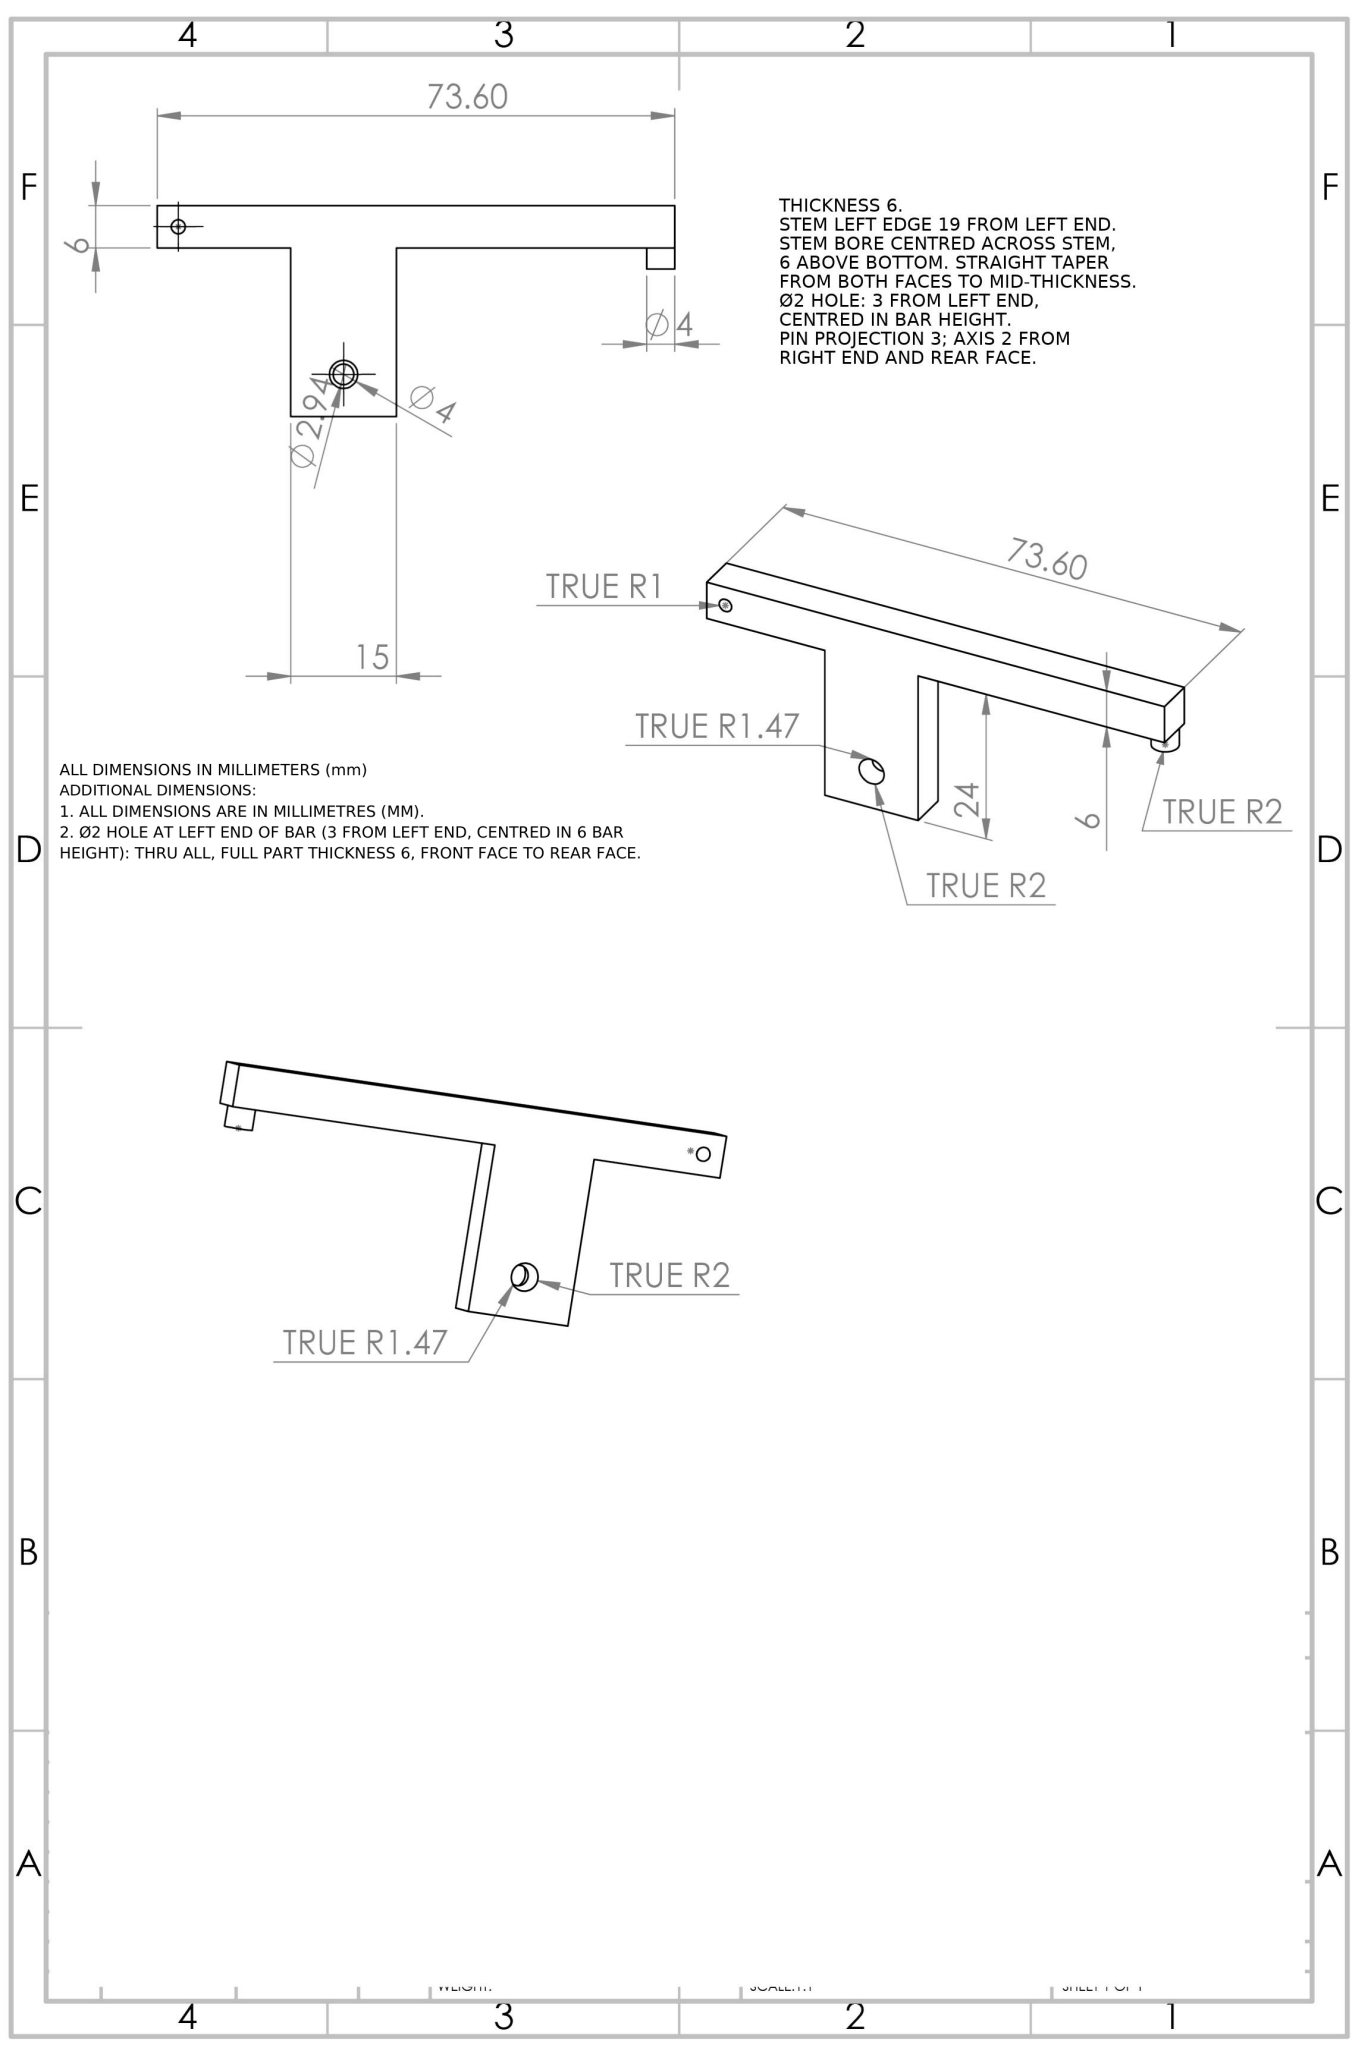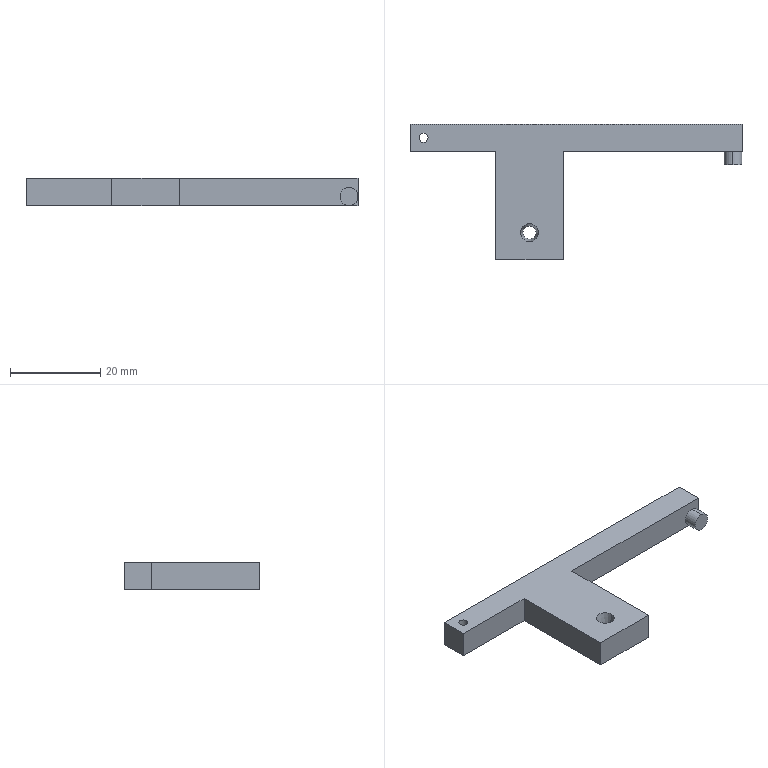Part | NX | mm | Z-Shaped Boss Link Bracket | 1 solid | 20 faces | box 73.6 x 30 x 6 mm | volume 4771 mm3 | plane 12 | cylinder 4 | cone 4 | commonest cylinder face diameters 4 x2 2 x2
STEP:
#1=COLOUR_RGB('',0.6706,0.8667,1.);
#2=FILL_AREA_STYLE_COLOUR('',#1);
#3=FILL_AREA_STYLE('',(#2));
#4=SURFACE_STYLE_FILL_AREA(#3);
#5=SURFACE_SIDE_STYLE('',(#4));
#6=SURFACE_STYLE_USAGE(.BOTH.,#5);
#7=PRESENTATION_STYLE_ASSIGNMENT((#6));
#8=CARTESIAN_POINT('',(2.,-9.,-0.));
#9=VERTEX_POINT('',#8);
#10=CARTESIAN_POINT('',(2.,-9.,4.));
#11=VERTEX_POINT('',#10);
#12=CARTESIAN_POINT('',(2.,-9.,2.));
#13=DIRECTION('',(0.,-1.,0.));
#14=DIRECTION('',(0.,0.,-1.));
#15=AXIS2_PLACEMENT_3D('',#12,#13,#14);
#16=CIRCLE('',#15,2.);
#17=EDGE_CURVE('',#9,#11,#16,.T.);
#18=ORIENTED_EDGE('',*,*,#17,.F.);
#19=CARTESIAN_POINT('',(2.,-6.,0.));
#20=VERTEX_POINT('',#19);
#21=CARTESIAN_POINT('',(2.,-9.,-0.));
#22=DIRECTION('',(0.,1.,0.));
#23=VECTOR('',#22,1000.);
#24=LINE('',#21,#23);
#25=EDGE_CURVE('',#9,#20,#24,.T.);
#26=ORIENTED_EDGE('',*,*,#25,.T.);
#27=CARTESIAN_POINT('',(4.,-6.,2.));
#28=VERTEX_POINT('',#27);
#29=CARTESIAN_POINT('',(2.,-6.,2.));
#30=DIRECTION('',(0.,-1.,0.));
#31=DIRECTION('',(0.,0.,-1.));
#32=AXIS2_PLACEMENT_3D('',#29,#30,#31);
#33=CIRCLE('',#32,2.);
#34=EDGE_CURVE('',#20,#28,#33,.T.);
#35=ORIENTED_EDGE('',*,*,#34,.T.);
#36=CARTESIAN_POINT('',(2.,-6.,4.));
#37=VERTEX_POINT('',#36);
#38=CARTESIAN_POINT('',(2.,-6.,2.));
#39=DIRECTION('',(0.,-1.,0.));
#40=DIRECTION('',(0.,0.,-1.));
#41=AXIS2_PLACEMENT_3D('',#38,#39,#40);
#42=CIRCLE('',#41,2.);
#43=EDGE_CURVE('',#28,#37,#42,.T.);
#44=ORIENTED_EDGE('',*,*,#43,.T.);
#45=CARTESIAN_POINT('',(2.,-9.,4.));
#46=DIRECTION('',(0.,1.,0.));
#47=VECTOR('',#46,1000.);
#48=LINE('',#45,#47);
#49=EDGE_CURVE('',#11,#37,#48,.T.);
#50=ORIENTED_EDGE('',*,*,#49,.F.);
#51=EDGE_LOOP('',(#18,#26,#35,#44,#50));
#52=FACE_OUTER_BOUND('',#51,.T.);
#53=CARTESIAN_POINT('',(2.,-9.,2.));
#54=DIRECTION('',(0.,1.,0.));
#55=DIRECTION('',(0.,0.,1.));
#56=AXIS2_PLACEMENT_3D('',#53,#54,#55);
#57=CYLINDRICAL_SURFACE('',#56,2.);
#58=ADVANCED_FACE('',(#52),#57,.T.);
#59=CARTESIAN_POINT('',(-67.6,-3.,0.));
#60=VERTEX_POINT('',#59);
#61=CARTESIAN_POINT('',(-65.6,-3.,0.));
#62=VERTEX_POINT('',#61);
#63=CARTESIAN_POINT('',(-66.6,-3.,0.));
#64=DIRECTION('',(0.,0.,1.));
#65=DIRECTION('',(1.,0.,0.));
#66=AXIS2_PLACEMENT_3D('',#63,#64,#65);
#67=CIRCLE('',#66,1.);
#68=EDGE_CURVE('',#60,#62,#67,.T.);
#69=ORIENTED_EDGE('',*,*,#68,.F.);
#70=CARTESIAN_POINT('',(-67.6,-3.,6.));
#71=VERTEX_POINT('',#70);
#72=CARTESIAN_POINT('',(-67.6,-3.,0.));
#73=DIRECTION('',(0.,0.,1.));
#74=VECTOR('',#73,1000.);
#75=LINE('',#72,#74);
#76=EDGE_CURVE('',#60,#71,#75,.T.);
#77=ORIENTED_EDGE('',*,*,#76,.T.);
#78=CARTESIAN_POINT('',(-65.6,-3.,6.));
#79=VERTEX_POINT('',#78);
#80=CARTESIAN_POINT('',(-66.6,-3.,6.));
#81=DIRECTION('',(0.,0.,1.));
#82=DIRECTION('',(1.,0.,0.));
#83=AXIS2_PLACEMENT_3D('',#80,#81,#82);
#84=CIRCLE('',#83,1.);
#85=EDGE_CURVE('',#71,#79,#84,.T.);
#86=ORIENTED_EDGE('',*,*,#85,.T.);
#87=CARTESIAN_POINT('',(-65.6,-3.,0.));
#88=DIRECTION('',(0.,0.,1.));
#89=VECTOR('',#88,1000.);
#90=LINE('',#87,#89);
#91=EDGE_CURVE('',#62,#79,#90,.T.);
#92=ORIENTED_EDGE('',*,*,#91,.F.);
#93=EDGE_LOOP('',(#69,#77,#86,#92));
#94=FACE_OUTER_BOUND('',#93,.T.);
#95=CARTESIAN_POINT('',(-66.6,-3.,0.));
#96=DIRECTION('',(0.,0.,1.));
#97=DIRECTION('',(1.,0.,0.));
#98=AXIS2_PLACEMENT_3D('',#95,#96,#97);
#99=CYLINDRICAL_SURFACE('',#98,1.);
#100=ADVANCED_FACE('',(#94),#99,.F.);
#101=CARTESIAN_POINT('',(-41.629,-24.,3.));
#102=VERTEX_POINT('',#101);
#103=CARTESIAN_POINT('',(-44.571,-24.,3.));
#104=VERTEX_POINT('',#103);
#105=CARTESIAN_POINT('',(-43.1,-24.,3.));
#106=DIRECTION('',(0.,0.,-1.));
#107=DIRECTION('',(-1.,0.,0.));
#108=AXIS2_PLACEMENT_3D('',#105,#106,#107);
#109=CIRCLE('',#108,1.471);
#110=EDGE_CURVE('',#102,#104,#109,.T.);
#111=ORIENTED_EDGE('',*,*,#110,.F.);
#112=CARTESIAN_POINT('',(-41.1,-24.,0.));
#113=VERTEX_POINT('',#112);
#114=CARTESIAN_POINT('',(-41.1,-24.,0.));
#115=DIRECTION('',(0.1736,0.,-0.9848));
#116=VECTOR('',#115,1000.);
#117=LINE('',#114,#116);
#118=EDGE_CURVE('',#102,#113,#117,.T.);
#119=ORIENTED_EDGE('',*,*,#118,.T.);
#120=CARTESIAN_POINT('',(-45.1,-24.,0.));
#121=VERTEX_POINT('',#120);
#122=CARTESIAN_POINT('',(-43.1,-24.,0.));
#123=DIRECTION('',(0.,0.,-1.));
#124=DIRECTION('',(-1.,0.,0.));
#125=AXIS2_PLACEMENT_3D('',#122,#123,#124);
#126=CIRCLE('',#125,2.);
#127=EDGE_CURVE('',#113,#121,#126,.T.);
#128=ORIENTED_EDGE('',*,*,#127,.T.);
#129=CARTESIAN_POINT('',(-45.1,-24.,0.));
#130=DIRECTION('',(-0.1736,0.,-0.9848));
#131=VECTOR('',#130,1000.);
#132=LINE('',#129,#131);
#133=EDGE_CURVE('',#104,#121,#132,.T.);
#134=ORIENTED_EDGE('',*,*,#133,.F.);
#135=EDGE_LOOP('',(#111,#119,#128,#134));
#136=FACE_OUTER_BOUND('',#135,.T.);
#137=CARTESIAN_POINT('',(-43.1,-24.,0.));
#138=DIRECTION('',(0.,0.,-1.));
#139=DIRECTION('',(-1.,0.,0.));
#140=AXIS2_PLACEMENT_3D('',#137,#138,#139);
#141=CONICAL_SURFACE('',#140,2.,0.1745);
#142=ADVANCED_FACE('',(#136),#141,.F.);
#143=ORIENTED_EDGE('',*,*,#110,.T.);
#144=CARTESIAN_POINT('',(-45.1,-24.,6.));
#145=VERTEX_POINT('',#144);
#146=CARTESIAN_POINT('',(-45.1,-24.,6.));
#147=DIRECTION('',(-0.1736,0.,0.9848));
#148=VECTOR('',#147,1000.);
#149=LINE('',#146,#148);
#150=EDGE_CURVE('',#104,#145,#149,.T.);
#151=ORIENTED_EDGE('',*,*,#150,.T.);
#152=CARTESIAN_POINT('',(-41.1,-24.,6.));
#153=VERTEX_POINT('',#152);
#154=CARTESIAN_POINT('',(-43.1,-24.,6.));
#155=DIRECTION('',(0.,0.,1.));
#156=DIRECTION('',(1.,0.,0.));
#157=AXIS2_PLACEMENT_3D('',#154,#155,#156);
#158=CIRCLE('',#157,2.);
#159=EDGE_CURVE('',#145,#153,#158,.T.);
#160=ORIENTED_EDGE('',*,*,#159,.T.);
#161=CARTESIAN_POINT('',(-41.1,-24.,6.));
#162=DIRECTION('',(0.1736,0.,0.9848));
#163=VECTOR('',#162,1000.);
#164=LINE('',#161,#163);
#165=EDGE_CURVE('',#102,#153,#164,.T.);
#166=ORIENTED_EDGE('',*,*,#165,.F.);
#167=EDGE_LOOP('',(#143,#151,#160,#166));
#168=FACE_OUTER_BOUND('',#167,.T.);
#169=CARTESIAN_POINT('',(-43.1,-24.,6.));
#170=DIRECTION('',(0.,0.,1.));
#171=DIRECTION('',(1.,0.,0.));
#172=AXIS2_PLACEMENT_3D('',#169,#170,#171);
#173=CONICAL_SURFACE('',#172,2.,0.1745);
#174=ADVANCED_FACE('',(#168),#173,.F.);
#175=ORIENTED_EDGE('',*,*,#34,.F.);
#176=CARTESIAN_POINT('',(4.,-6.,0.));
#177=VERTEX_POINT('',#176);
#178=CARTESIAN_POINT('',(0.,-6.,0.));
#179=DIRECTION('',(1.,0.,0.));
#180=VECTOR('',#179,1000.);
#181=LINE('',#178,#180);
#182=EDGE_CURVE('',#20,#177,#181,.T.);
#183=ORIENTED_EDGE('',*,*,#182,.T.);
#184=CARTESIAN_POINT('',(4.,-6.,6.));
#185=DIRECTION('',(0.,0.,-1.));
#186=VECTOR('',#185,1000.);
#187=LINE('',#184,#186);
#188=EDGE_CURVE('',#28,#177,#187,.T.);
#189=ORIENTED_EDGE('',*,*,#188,.F.);
#190=EDGE_LOOP('',(#175,#183,#189));
#191=FACE_OUTER_BOUND('',#190,.T.);
#192=CARTESIAN_POINT('',(0.,-6.,6.));
#193=DIRECTION('',(0.,1.,0.));
#194=DIRECTION('',(0.,0.,1.));
#195=AXIS2_PLACEMENT_3D('',#192,#193,#194);
#196=PLANE('',#195);
#197=ADVANCED_FACE('',(#191),#196,.F.);
#198=CARTESIAN_POINT('',(4.,-0.,0.));
#199=VERTEX_POINT('',#198);
#200=CARTESIAN_POINT('',(-69.6,-0.,0.));
#201=VERTEX_POINT('',#200);
#202=CARTESIAN_POINT('',(-69.6,-0.,0.));
#203=DIRECTION('',(-1.,-0.,0.));
#204=VECTOR('',#203,1000.);
#205=LINE('',#202,#204);
#206=EDGE_CURVE('',#199,#201,#205,.T.);
#207=ORIENTED_EDGE('',*,*,#206,.T.);
#208=CARTESIAN_POINT('',(-69.6,-0.,6.));
#209=VERTEX_POINT('',#208);
#210=CARTESIAN_POINT('',(-69.6,-0.,6.));
#211=DIRECTION('',(0.,0.,-1.));
#212=VECTOR('',#211,1000.);
#213=LINE('',#210,#212);
#214=EDGE_CURVE('',#209,#201,#213,.T.);
#215=ORIENTED_EDGE('',*,*,#214,.F.);
#216=CARTESIAN_POINT('',(4.,-0.,6.));
#217=VERTEX_POINT('',#216);
#218=CARTESIAN_POINT('',(-69.6,-0.,6.));
#219=DIRECTION('',(-1.,-0.,0.));
#220=VECTOR('',#219,1000.);
#221=LINE('',#218,#220);
#222=EDGE_CURVE('',#217,#209,#221,.T.);
#223=ORIENTED_EDGE('',*,*,#222,.F.);
#224=CARTESIAN_POINT('',(4.,-0.,6.));
#225=DIRECTION('',(0.,0.,-1.));
#226=VECTOR('',#225,1000.);
#227=LINE('',#224,#226);
#228=EDGE_CURVE('',#217,#199,#227,.T.);
#229=ORIENTED_EDGE('',*,*,#228,.T.);
#230=EDGE_LOOP('',(#207,#215,#223,#229));
#231=FACE_OUTER_BOUND('',#230,.T.);
#232=CARTESIAN_POINT('',(-69.6,-0.,6.));
#233=DIRECTION('',(0.,-1.,0.));
#234=DIRECTION('',(1.,0.,0.));
#235=AXIS2_PLACEMENT_3D('',#232,#233,#234);
#236=PLANE('',#235);
#237=ADVANCED_FACE('',(#231),#236,.F.);
#238=CARTESIAN_POINT('',(-69.6,-6.,0.));
#239=VERTEX_POINT('',#238);
#240=CARTESIAN_POINT('',(-69.6,-0.,0.));
#241=DIRECTION('',(0.,-1.,0.));
#242=VECTOR('',#241,1000.);
#243=LINE('',#240,#242);
#244=EDGE_CURVE('',#201,#239,#243,.T.);
#245=ORIENTED_EDGE('',*,*,#244,.T.);
#246=CARTESIAN_POINT('',(-69.6,-6.,6.));
#247=VERTEX_POINT('',#246);
#248=CARTESIAN_POINT('',(-69.6,-6.,6.));
#249=DIRECTION('',(0.,0.,-1.));
#250=VECTOR('',#249,1000.);
#251=LINE('',#248,#250);
#252=EDGE_CURVE('',#247,#239,#251,.T.);
#253=ORIENTED_EDGE('',*,*,#252,.F.);
#254=CARTESIAN_POINT('',(-69.6,-0.,6.));
#255=DIRECTION('',(0.,-1.,0.));
#256=VECTOR('',#255,1000.);
#257=LINE('',#254,#256);
#258=EDGE_CURVE('',#209,#247,#257,.T.);
#259=ORIENTED_EDGE('',*,*,#258,.F.);
#260=ORIENTED_EDGE('',*,*,#214,.T.);
#261=EDGE_LOOP('',(#245,#253,#259,#260));
#262=FACE_OUTER_BOUND('',#261,.T.);
#263=CARTESIAN_POINT('',(-69.6,-0.,6.));
#264=DIRECTION('',(1.,0.,0.));
#265=DIRECTION('',(0.,0.,-1.));
#266=AXIS2_PLACEMENT_3D('',#263,#264,#265);
#267=PLANE('',#266);
#268=ADVANCED_FACE('',(#262),#267,.F.);
#269=CARTESIAN_POINT('',(-50.6,-6.,0.));
#270=VERTEX_POINT('',#269);
#271=CARTESIAN_POINT('',(-69.6,-6.,0.));
#272=DIRECTION('',(1.,0.,0.));
#273=VECTOR('',#272,1000.);
#274=LINE('',#271,#273);
#275=EDGE_CURVE('',#239,#270,#274,.T.);
#276=ORIENTED_EDGE('',*,*,#275,.T.);
#277=CARTESIAN_POINT('',(-50.6,-6.,6.));
#278=VERTEX_POINT('',#277);
#279=CARTESIAN_POINT('',(-50.6,-6.,6.));
#280=DIRECTION('',(0.,0.,-1.));
#281=VECTOR('',#280,1000.);
#282=LINE('',#279,#281);
#283=EDGE_CURVE('',#278,#270,#282,.T.);
#284=ORIENTED_EDGE('',*,*,#283,.F.);
#285=CARTESIAN_POINT('',(-69.6,-6.,6.));
#286=DIRECTION('',(1.,0.,0.));
#287=VECTOR('',#286,1000.);
#288=LINE('',#285,#287);
#289=EDGE_CURVE('',#247,#278,#288,.T.);
#290=ORIENTED_EDGE('',*,*,#289,.F.);
#291=ORIENTED_EDGE('',*,*,#252,.T.);
#292=EDGE_LOOP('',(#276,#284,#290,#291));
#293=FACE_OUTER_BOUND('',#292,.T.);
#294=CARTESIAN_POINT('',(-69.6,-6.,6.));
#295=DIRECTION('',(-0.,1.,0.));
#296=DIRECTION('',(-1.,-0.,0.));
#297=AXIS2_PLACEMENT_3D('',#294,#295,#296);
#298=PLANE('',#297);
#299=ADVANCED_FACE('',(#293),#298,.F.);
#300=CARTESIAN_POINT('',(-50.6,-30.,0.));
#301=VERTEX_POINT('',#300);
#302=CARTESIAN_POINT('',(-50.6,-6.,0.));
#303=DIRECTION('',(0.,-1.,0.));
#304=VECTOR('',#303,1000.);
#305=LINE('',#302,#304);
#306=EDGE_CURVE('',#270,#301,#305,.T.);
#307=ORIENTED_EDGE('',*,*,#306,.T.);
#308=CARTESIAN_POINT('',(-50.6,-30.,6.));
#309=VERTEX_POINT('',#308);
#310=CARTESIAN_POINT('',(-50.6,-30.,6.));
#311=DIRECTION('',(0.,0.,-1.));
#312=VECTOR('',#311,1000.);
#313=LINE('',#310,#312);
#314=EDGE_CURVE('',#309,#301,#313,.T.);
#315=ORIENTED_EDGE('',*,*,#314,.F.);
#316=CARTESIAN_POINT('',(-50.6,-6.,6.));
#317=DIRECTION('',(0.,-1.,0.));
#318=VECTOR('',#317,1000.);
#319=LINE('',#316,#318);
#320=EDGE_CURVE('',#278,#309,#319,.T.);
#321=ORIENTED_EDGE('',*,*,#320,.F.);
#322=ORIENTED_EDGE('',*,*,#283,.T.);
#323=EDGE_LOOP('',(#307,#315,#321,#322));
#324=FACE_OUTER_BOUND('',#323,.T.);
#325=CARTESIAN_POINT('',(-50.6,-6.,6.));
#326=DIRECTION('',(1.,0.,0.));
#327=DIRECTION('',(-0.,1.,0.));
#328=AXIS2_PLACEMENT_3D('',#325,#326,#327);
#329=PLANE('',#328);
#330=ADVANCED_FACE('',(#324),#329,.F.);
#331=CARTESIAN_POINT('',(-35.6,-30.,0.));
#332=VERTEX_POINT('',#331);
#333=CARTESIAN_POINT('',(-50.6,-30.,0.));
#334=DIRECTION('',(1.,0.,0.));
#335=VECTOR('',#334,1000.);
#336=LINE('',#333,#335);
#337=EDGE_CURVE('',#301,#332,#336,.T.);
#338=ORIENTED_EDGE('',*,*,#337,.T.);
#339=CARTESIAN_POINT('',(-35.6,-30.,6.));
#340=VERTEX_POINT('',#339);
#341=CARTESIAN_POINT('',(-35.6,-30.,6.));
#342=DIRECTION('',(0.,0.,-1.));
#343=VECTOR('',#342,1000.);
#344=LINE('',#341,#343);
#345=EDGE_CURVE('',#340,#332,#344,.T.);
#346=ORIENTED_EDGE('',*,*,#345,.F.);
#347=CARTESIAN_POINT('',(-50.6,-30.,6.));
#348=DIRECTION('',(1.,0.,0.));
#349=VECTOR('',#348,1000.);
#350=LINE('',#347,#349);
#351=EDGE_CURVE('',#309,#340,#350,.T.);
#352=ORIENTED_EDGE('',*,*,#351,.F.);
#353=ORIENTED_EDGE('',*,*,#314,.T.);
#354=EDGE_LOOP('',(#338,#346,#352,#353));
#355=FACE_OUTER_BOUND('',#354,.T.);
#356=CARTESIAN_POINT('',(-50.6,-30.,6.));
#357=DIRECTION('',(0.,1.,0.));
#358=DIRECTION('',(0.,0.,1.));
#359=AXIS2_PLACEMENT_3D('',#356,#357,#358);
#360=PLANE('',#359);
#361=ADVANCED_FACE('',(#355),#360,.F.);
#362=CARTESIAN_POINT('',(-35.6,-6.,0.));
#363=VERTEX_POINT('',#362);
#364=CARTESIAN_POINT('',(-35.6,-30.,0.));
#365=DIRECTION('',(0.,1.,0.));
#366=VECTOR('',#365,1000.);
#367=LINE('',#364,#366);
#368=EDGE_CURVE('',#332,#363,#367,.T.);
#369=ORIENTED_EDGE('',*,*,#368,.T.);
#370=CARTESIAN_POINT('',(-35.6,-6.,6.));
#371=VERTEX_POINT('',#370);
#372=CARTESIAN_POINT('',(-35.6,-6.,6.));
#373=DIRECTION('',(0.,0.,-1.));
#374=VECTOR('',#373,1000.);
#375=LINE('',#372,#374);
#376=EDGE_CURVE('',#371,#363,#375,.T.);
#377=ORIENTED_EDGE('',*,*,#376,.F.);
#378=CARTESIAN_POINT('',(-35.6,-30.,6.));
#379=DIRECTION('',(0.,1.,0.));
#380=VECTOR('',#379,1000.);
#381=LINE('',#378,#380);
#382=EDGE_CURVE('',#340,#371,#381,.T.);
#383=ORIENTED_EDGE('',*,*,#382,.F.);
#384=ORIENTED_EDGE('',*,*,#345,.T.);
#385=EDGE_LOOP('',(#369,#377,#383,#384));
#386=FACE_OUTER_BOUND('',#385,.T.);
#387=CARTESIAN_POINT('',(-35.6,-30.,6.));
#388=DIRECTION('',(-1.,0.,0.));
#389=DIRECTION('',(0.,0.,1.));
#390=AXIS2_PLACEMENT_3D('',#387,#388,#389);
#391=PLANE('',#390);
#392=ADVANCED_FACE('',(#386),#391,.F.);
#393=ORIENTED_EDGE('',*,*,#43,.F.);
#394=CARTESIAN_POINT('',(4.,-6.,6.));
#395=VERTEX_POINT('',#394);
#396=CARTESIAN_POINT('',(4.,-6.,6.));
#397=DIRECTION('',(0.,0.,-1.));
#398=VECTOR('',#397,1000.);
#399=LINE('',#396,#398);
#400=EDGE_CURVE('',#395,#28,#399,.T.);
#401=ORIENTED_EDGE('',*,*,#400,.F.);
#402=CARTESIAN_POINT('',(-35.6,-6.,6.));
#403=DIRECTION('',(1.,0.,0.));
#404=VECTOR('',#403,1000.);
#405=LINE('',#402,#404);
#406=EDGE_CURVE('',#371,#395,#405,.T.);
#407=ORIENTED_EDGE('',*,*,#406,.F.);
#408=ORIENTED_EDGE('',*,*,#376,.T.);
#409=CARTESIAN_POINT('',(0.,-6.,0.));
#410=DIRECTION('',(1.,0.,0.));
#411=VECTOR('',#410,1000.);
#412=LINE('',#409,#411);
#413=EDGE_CURVE('',#363,#20,#412,.T.);
#414=ORIENTED_EDGE('',*,*,#413,.T.);
#415=CARTESIAN_POINT('',(2.,-6.,2.));
#416=DIRECTION('',(0.,-1.,0.));
#417=DIRECTION('',(0.,0.,-1.));
#418=AXIS2_PLACEMENT_3D('',#415,#416,#417);
#419=CIRCLE('',#418,2.);
#420=EDGE_CURVE('',#37,#20,#419,.T.);
#421=ORIENTED_EDGE('',*,*,#420,.F.);
#422=EDGE_LOOP('',(#393,#401,#407,#408,#414,#421));
#423=FACE_OUTER_BOUND('',#422,.T.);
#424=CARTESIAN_POINT('',(0.,-6.,6.));
#425=DIRECTION('',(0.,1.,0.));
#426=DIRECTION('',(0.,0.,1.));
#427=AXIS2_PLACEMENT_3D('',#424,#425,#426);
#428=PLANE('',#427);
#429=ADVANCED_FACE('',(#423),#428,.F.);
#430=CARTESIAN_POINT('',(4.,-6.,0.));
#431=DIRECTION('',(-0.,1.,0.));
#432=VECTOR('',#431,1000.);
#433=LINE('',#430,#432);
#434=EDGE_CURVE('',#177,#199,#433,.T.);
#435=ORIENTED_EDGE('',*,*,#434,.T.);
#436=ORIENTED_EDGE('',*,*,#228,.F.);
#437=CARTESIAN_POINT('',(4.,-6.,6.));
#438=DIRECTION('',(-0.,1.,0.));
#439=VECTOR('',#438,1000.);
#440=LINE('',#437,#439);
#441=EDGE_CURVE('',#395,#217,#440,.T.);
#442=ORIENTED_EDGE('',*,*,#441,.F.);
#443=ORIENTED_EDGE('',*,*,#400,.T.);
#444=ORIENTED_EDGE('',*,*,#188,.T.);
#445=EDGE_LOOP('',(#435,#436,#442,#443,#444));
#446=FACE_OUTER_BOUND('',#445,.T.);
#447=CARTESIAN_POINT('',(4.,-6.,6.));
#448=DIRECTION('',(-1.,-0.,0.));
#449=DIRECTION('',(0.,-1.,0.));
#450=AXIS2_PLACEMENT_3D('',#447,#448,#449);
#451=PLANE('',#450);
#452=ADVANCED_FACE('',(#446),#451,.F.);
#453=CARTESIAN_POINT('',(-66.6,-3.,6.));
#454=DIRECTION('',(0.,0.,1.));
#455=DIRECTION('',(1.,0.,0.));
#456=AXIS2_PLACEMENT_3D('',#453,#454,#455);
#457=CIRCLE('',#456,1.);
#458=EDGE_CURVE('',#79,#71,#457,.T.);
#459=ORIENTED_EDGE('',*,*,#458,.F.);
#460=ORIENTED_EDGE('',*,*,#85,.F.);
#461=EDGE_LOOP('',(#459,#460));
#462=FACE_BOUND('',#461,.T.);
#463=CARTESIAN_POINT('',(-43.1,-24.,6.));
#464=DIRECTION('',(0.,0.,1.));
#465=DIRECTION('',(1.,0.,0.));
#466=AXIS2_PLACEMENT_3D('',#463,#464,#465);
#467=CIRCLE('',#466,2.);
#468=EDGE_CURVE('',#153,#145,#467,.T.);
#469=ORIENTED_EDGE('',*,*,#468,.F.);
#470=ORIENTED_EDGE('',*,*,#159,.F.);
#471=EDGE_LOOP('',(#469,#470));
#472=FACE_BOUND('',#471,.T.);
#473=ORIENTED_EDGE('',*,*,#222,.T.);
#474=ORIENTED_EDGE('',*,*,#258,.T.);
#475=ORIENTED_EDGE('',*,*,#289,.T.);
#476=ORIENTED_EDGE('',*,*,#320,.T.);
#477=ORIENTED_EDGE('',*,*,#351,.T.);
#478=ORIENTED_EDGE('',*,*,#382,.T.);
#479=ORIENTED_EDGE('',*,*,#406,.T.);
#480=ORIENTED_EDGE('',*,*,#441,.T.);
#481=EDGE_LOOP('',(#473,#474,#475,#476,#477,#478,#479,#480));
#482=FACE_OUTER_BOUND('',#481,.T.);
#483=CARTESIAN_POINT('',(0.,0.,6.));
#484=DIRECTION('',(0.,0.,1.));
#485=DIRECTION('',(1.,0.,0.));
#486=AXIS2_PLACEMENT_3D('',#483,#484,#485);
#487=PLANE('',#486);
#488=ADVANCED_FACE('',(#462,#472,#482),#487,.T.);
#489=CARTESIAN_POINT('',(-66.6,-3.,0.));
#490=DIRECTION('',(0.,0.,1.));
#491=DIRECTION('',(1.,0.,0.));
#492=AXIS2_PLACEMENT_3D('',#489,#490,#491);
#493=CIRCLE('',#492,1.);
#494=EDGE_CURVE('',#62,#60,#493,.T.);
#495=ORIENTED_EDGE('',*,*,#494,.T.);
#496=ORIENTED_EDGE('',*,*,#68,.T.);
#497=EDGE_LOOP('',(#495,#496));
#498=FACE_BOUND('',#497,.T.);
#499=CARTESIAN_POINT('',(-43.1,-24.,0.));
#500=DIRECTION('',(0.,0.,-1.));
#501=DIRECTION('',(-1.,0.,0.));
#502=AXIS2_PLACEMENT_3D('',#499,#500,#501);
#503=CIRCLE('',#502,2.);
#504=EDGE_CURVE('',#121,#113,#503,.T.);
#505=ORIENTED_EDGE('',*,*,#504,.F.);
#506=ORIENTED_EDGE('',*,*,#127,.F.);
#507=EDGE_LOOP('',(#505,#506));
#508=FACE_BOUND('',#507,.T.);
#509=ORIENTED_EDGE('',*,*,#206,.F.);
#510=ORIENTED_EDGE('',*,*,#434,.F.);
#511=ORIENTED_EDGE('',*,*,#182,.F.);
#512=ORIENTED_EDGE('',*,*,#413,.F.);
#513=ORIENTED_EDGE('',*,*,#368,.F.);
#514=ORIENTED_EDGE('',*,*,#337,.F.);
#515=ORIENTED_EDGE('',*,*,#306,.F.);
#516=ORIENTED_EDGE('',*,*,#275,.F.);
#517=ORIENTED_EDGE('',*,*,#244,.F.);
#518=EDGE_LOOP('',(#509,#510,#511,#512,#513,#514,#515,#516,#517));
#519=FACE_OUTER_BOUND('',#518,.T.);
#520=CARTESIAN_POINT('',(0.,0.,0.));
#521=DIRECTION('',(0.,0.,1.));
#522=DIRECTION('',(1.,0.,0.));
#523=AXIS2_PLACEMENT_3D('',#520,#521,#522);
#524=PLANE('',#523);
#525=ADVANCED_FACE('',(#498,#508,#519),#524,.F.);
#526=ORIENTED_EDGE('',*,*,#150,.F.);
#527=CARTESIAN_POINT('',(-43.1,-24.,3.));
#528=DIRECTION('',(0.,0.,-1.));
#529=DIRECTION('',(-1.,0.,0.));
#530=AXIS2_PLACEMENT_3D('',#527,#528,#529);
#531=CIRCLE('',#530,1.471);
#532=EDGE_CURVE('',#104,#102,#531,.T.);
#533=ORIENTED_EDGE('',*,*,#532,.T.);
#534=ORIENTED_EDGE('',*,*,#165,.T.);
#535=ORIENTED_EDGE('',*,*,#468,.T.);
#536=EDGE_LOOP('',(#526,#533,#534,#535));
#537=FACE_OUTER_BOUND('',#536,.T.);
#538=CARTESIAN_POINT('',(-43.1,-24.,6.));
#539=DIRECTION('',(0.,0.,1.));
#540=DIRECTION('',(1.,0.,0.));
#541=AXIS2_PLACEMENT_3D('',#538,#539,#540);
#542=CONICAL_SURFACE('',#541,2.,0.1745);
#543=ADVANCED_FACE('',(#537),#542,.F.);
#544=ORIENTED_EDGE('',*,*,#118,.F.);
#545=ORIENTED_EDGE('',*,*,#532,.F.);
#546=ORIENTED_EDGE('',*,*,#133,.T.);
#547=ORIENTED_EDGE('',*,*,#504,.T.);
#548=EDGE_LOOP('',(#544,#545,#546,#547));
#549=FACE_OUTER_BOUND('',#548,.T.);
#550=CARTESIAN_POINT('',(-43.1,-24.,0.));
#551=DIRECTION('',(0.,0.,-1.));
#552=DIRECTION('',(-1.,0.,0.));
#553=AXIS2_PLACEMENT_3D('',#550,#551,#552);
#554=CONICAL_SURFACE('',#553,2.,0.1745);
#555=ADVANCED_FACE('',(#549),#554,.F.);
#556=ORIENTED_EDGE('',*,*,#76,.F.);
#557=ORIENTED_EDGE('',*,*,#494,.F.);
#558=ORIENTED_EDGE('',*,*,#91,.T.);
#559=ORIENTED_EDGE('',*,*,#458,.T.);
#560=EDGE_LOOP('',(#556,#557,#558,#559));
#561=FACE_OUTER_BOUND('',#560,.T.);
#562=CARTESIAN_POINT('',(-66.6,-3.,0.));
#563=DIRECTION('',(0.,0.,1.));
#564=DIRECTION('',(1.,0.,0.));
#565=AXIS2_PLACEMENT_3D('',#562,#563,#564);
#566=CYLINDRICAL_SURFACE('',#565,1.);
#567=ADVANCED_FACE('',(#561),#566,.F.);
#568=ORIENTED_EDGE('',*,*,#25,.F.);
#569=CARTESIAN_POINT('',(2.,-9.,2.));
#570=DIRECTION('',(0.,-1.,0.));
#571=DIRECTION('',(0.,0.,-1.));
#572=AXIS2_PLACEMENT_3D('',#569,#570,#571);
#573=CIRCLE('',#572,2.);
#574=EDGE_CURVE('',#11,#9,#573,.T.);
#575=ORIENTED_EDGE('',*,*,#574,.F.);
#576=ORIENTED_EDGE('',*,*,#49,.T.);
#577=ORIENTED_EDGE('',*,*,#420,.T.);
#578=EDGE_LOOP('',(#568,#575,#576,#577));
#579=FACE_OUTER_BOUND('',#578,.T.);
#580=CARTESIAN_POINT('',(2.,-9.,2.));
#581=DIRECTION('',(0.,1.,0.));
#582=DIRECTION('',(0.,0.,1.));
#583=AXIS2_PLACEMENT_3D('',#580,#581,#582);
#584=CYLINDRICAL_SURFACE('',#583,2.);
#585=ADVANCED_FACE('',(#579),#584,.T.);
#586=ORIENTED_EDGE('',*,*,#574,.T.);
#587=ORIENTED_EDGE('',*,*,#17,.T.);
#588=EDGE_LOOP('',(#586,#587));
#589=FACE_OUTER_BOUND('',#588,.T.);
#590=CARTESIAN_POINT('',(2.,-9.,2.));
#591=DIRECTION('',(0.,-1.,0.));
#592=DIRECTION('',(0.,0.,-1.));
#593=AXIS2_PLACEMENT_3D('',#590,#591,#592);
#594=PLANE('',#593);
#595=ADVANCED_FACE('',(#589),#594,.T.);
#596=CLOSED_SHELL('',(#58,#100,#142,#174,#197,#237,#268,#299,#330,#361,#392,#429,#452,#488,#525,#543,#555,#567,#585,#595));
#597=MANIFOLD_SOLID_BREP('',#596);
#598=STYLED_ITEM('',(#7),#597);
#599=PRESENTATION_LAYER_ASSIGNMENT('','',(#598));
#600=(LENGTH_UNIT()NAMED_UNIT(*)SI_UNIT(.MILLI.,.METRE.));
#601=UNCERTAINTY_MEASURE_WITH_UNIT(LENGTH_MEASURE(0.00001),#600,'','');
#602=(NAMED_UNIT(*)PLANE_ANGLE_UNIT()SI_UNIT($,.RADIAN.));
#603=(NAMED_UNIT(*)SI_UNIT($,.STERADIAN.)SOLID_ANGLE_UNIT());
#604=(GEOMETRIC_REPRESENTATION_CONTEXT(3)GLOBAL_UNCERTAINTY_ASSIGNED_CONTEXT((#601))GLOBAL_UNIT_ASSIGNED_CONTEXT((#600,#602,#603))REPRESENTATION_CONTEXT('',''));
#605=MECHANICAL_DESIGN_GEOMETRIC_PRESENTATION_REPRESENTATION('',(#598),#604);
#606=COLOUR_RGB('',0.7922,0.8196,0.9333);
#607=FILL_AREA_STYLE_COLOUR('',#606);
#608=FILL_AREA_STYLE('',(#607));
#609=SURFACE_STYLE_FILL_AREA(#608);
#610=SURFACE_SIDE_STYLE('',(#609));
#611=SURFACE_STYLE_USAGE(.BOTH.,#610);
#612=PRESENTATION_STYLE_ASSIGNMENT((#611));
#613=CARTESIAN_POINT('',(0.,0.,0.));
#614=DIRECTION('',(0.,0.,1.));
#615=DIRECTION('',(1.,0.,0.));
#616=AXIS2_PLACEMENT_3D('',#613,#614,#615);
#617=(LENGTH_UNIT()NAMED_UNIT(*)SI_UNIT(.MILLI.,.METRE.));
#618=UNCERTAINTY_MEASURE_WITH_UNIT(LENGTH_MEASURE(0.00001),#617,'','');
#619=(NAMED_UNIT(*)PLANE_ANGLE_UNIT()SI_UNIT($,.RADIAN.));
#620=(NAMED_UNIT(*)SI_UNIT($,.STERADIAN.)SOLID_ANGLE_UNIT());
#621=(GEOMETRIC_REPRESENTATION_CONTEXT(3)GLOBAL_UNCERTAINTY_ASSIGNED_CONTEXT((#618))GLOBAL_UNIT_ASSIGNED_CONTEXT((#617,#619,#620))REPRESENTATION_CONTEXT('',''));
#622=ADVANCED_BREP_SHAPE_REPRESENTATION('',(#597,#616),#621);
#623=STYLED_ITEM('',(#612),#622);
#624=PRESENTATION_LAYER_ASSIGNMENT('','',(#623));
#625=(LENGTH_UNIT()NAMED_UNIT(*)SI_UNIT(.MILLI.,.METRE.));
#626=UNCERTAINTY_MEASURE_WITH_UNIT(LENGTH_MEASURE(0.00001),#625,'','');
#627=(NAMED_UNIT(*)PLANE_ANGLE_UNIT()SI_UNIT($,.RADIAN.));
#628=(NAMED_UNIT(*)SI_UNIT($,.STERADIAN.)SOLID_ANGLE_UNIT());
#629=(GEOMETRIC_REPRESENTATION_CONTEXT(3)GLOBAL_UNCERTAINTY_ASSIGNED_CONTEXT((#626))GLOBAL_UNIT_ASSIGNED_CONTEXT((#625,#627,#628))REPRESENTATION_CONTEXT('',''));
#630=MECHANICAL_DESIGN_GEOMETRIC_PRESENTATION_REPRESENTATION('',(#623),#629);